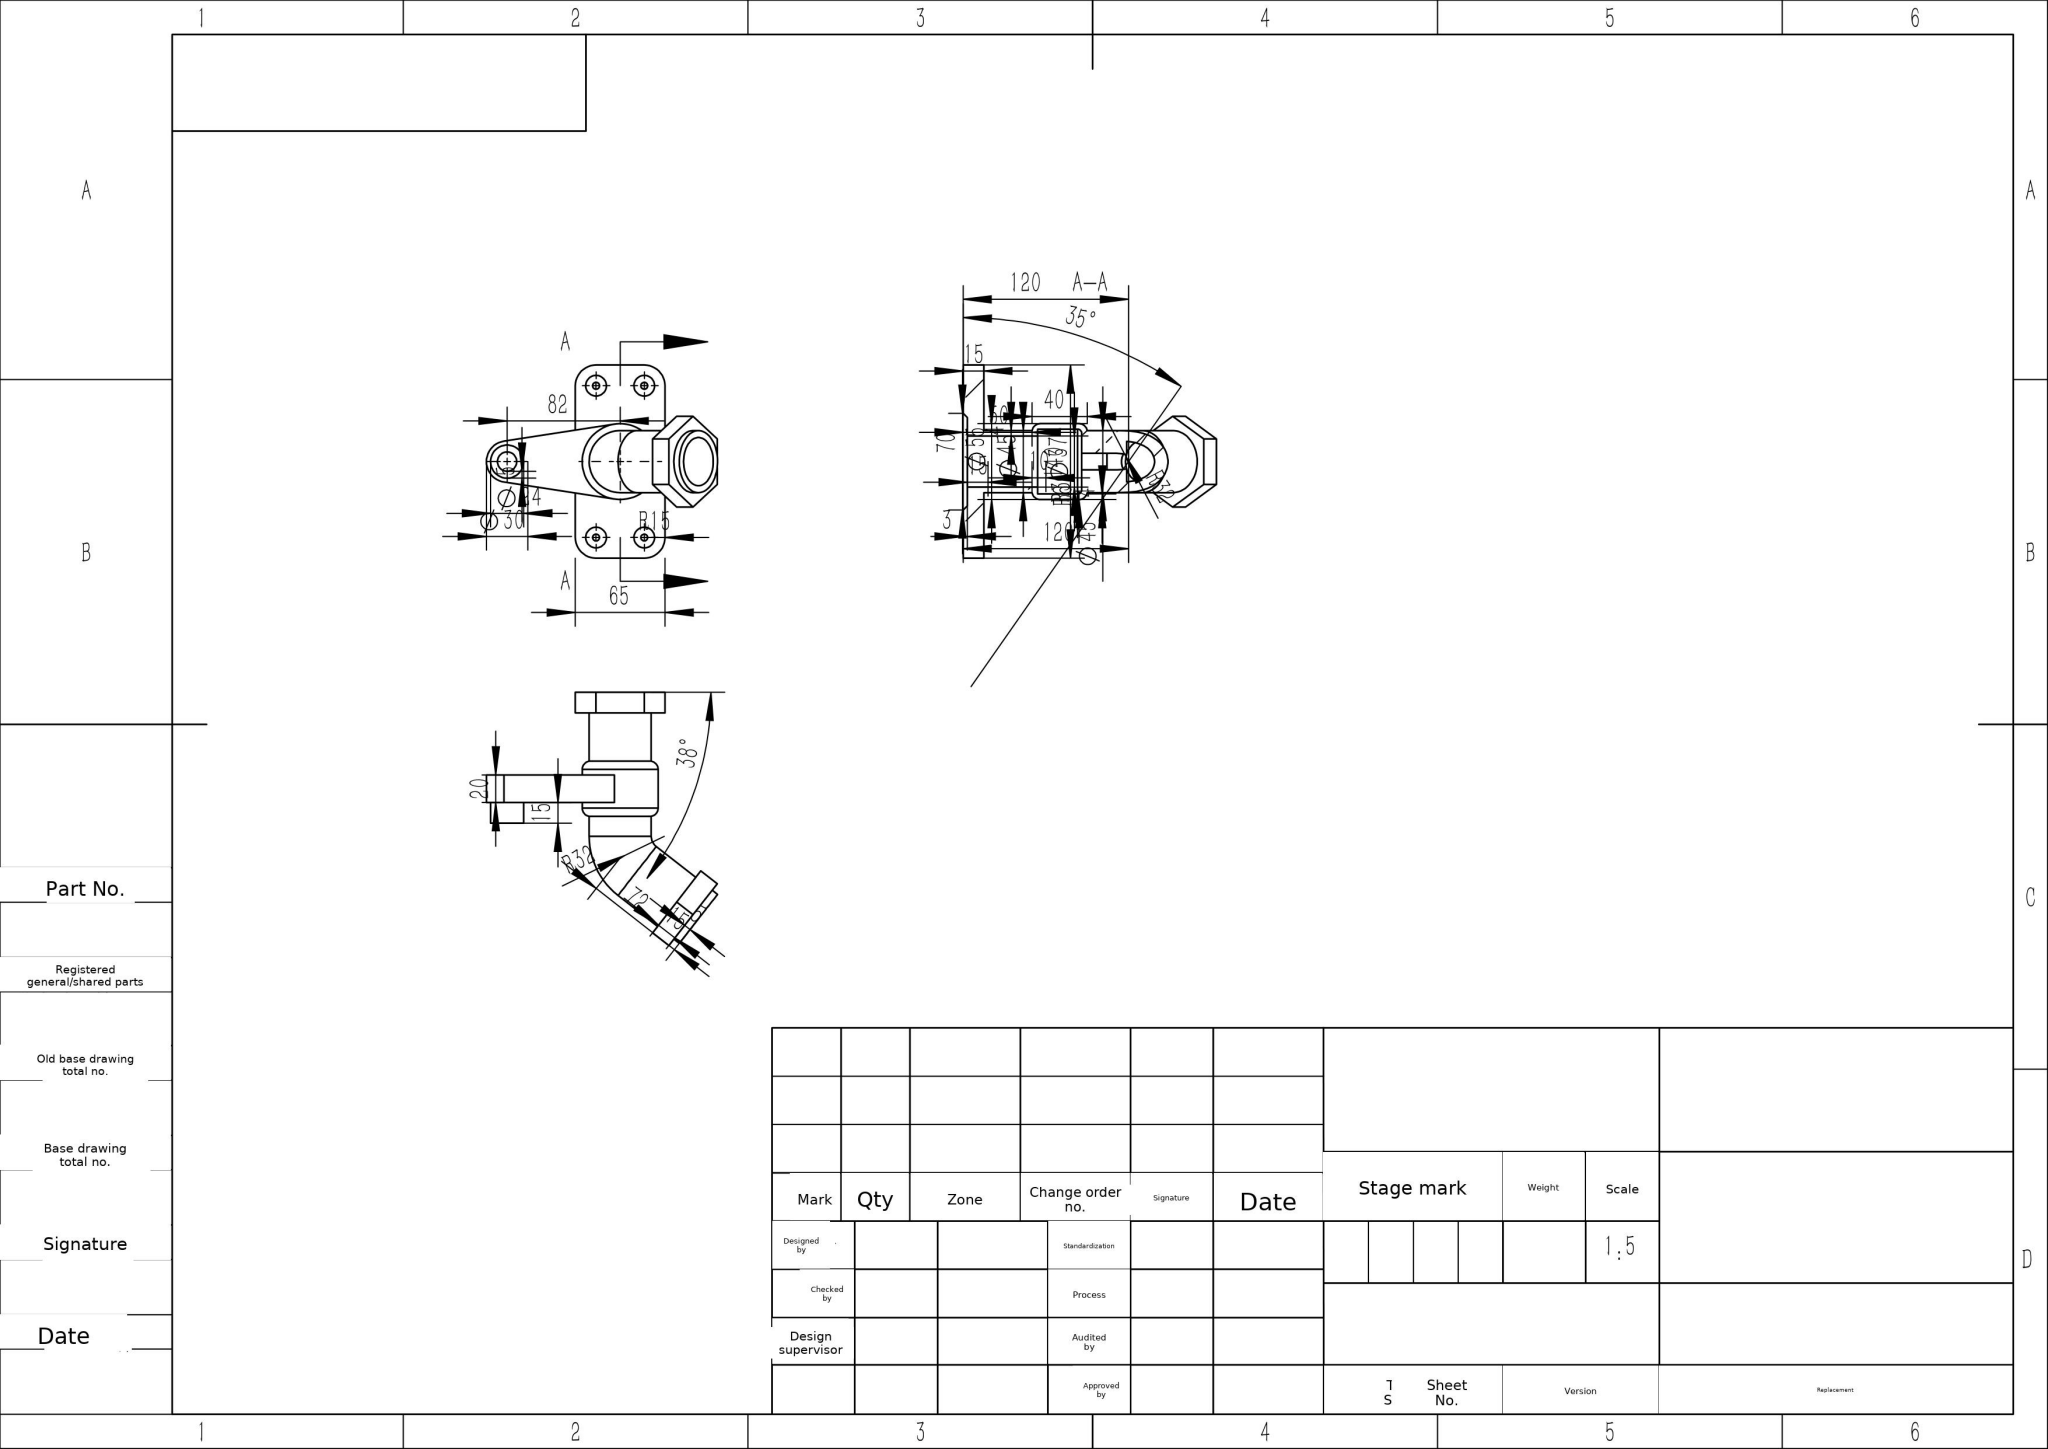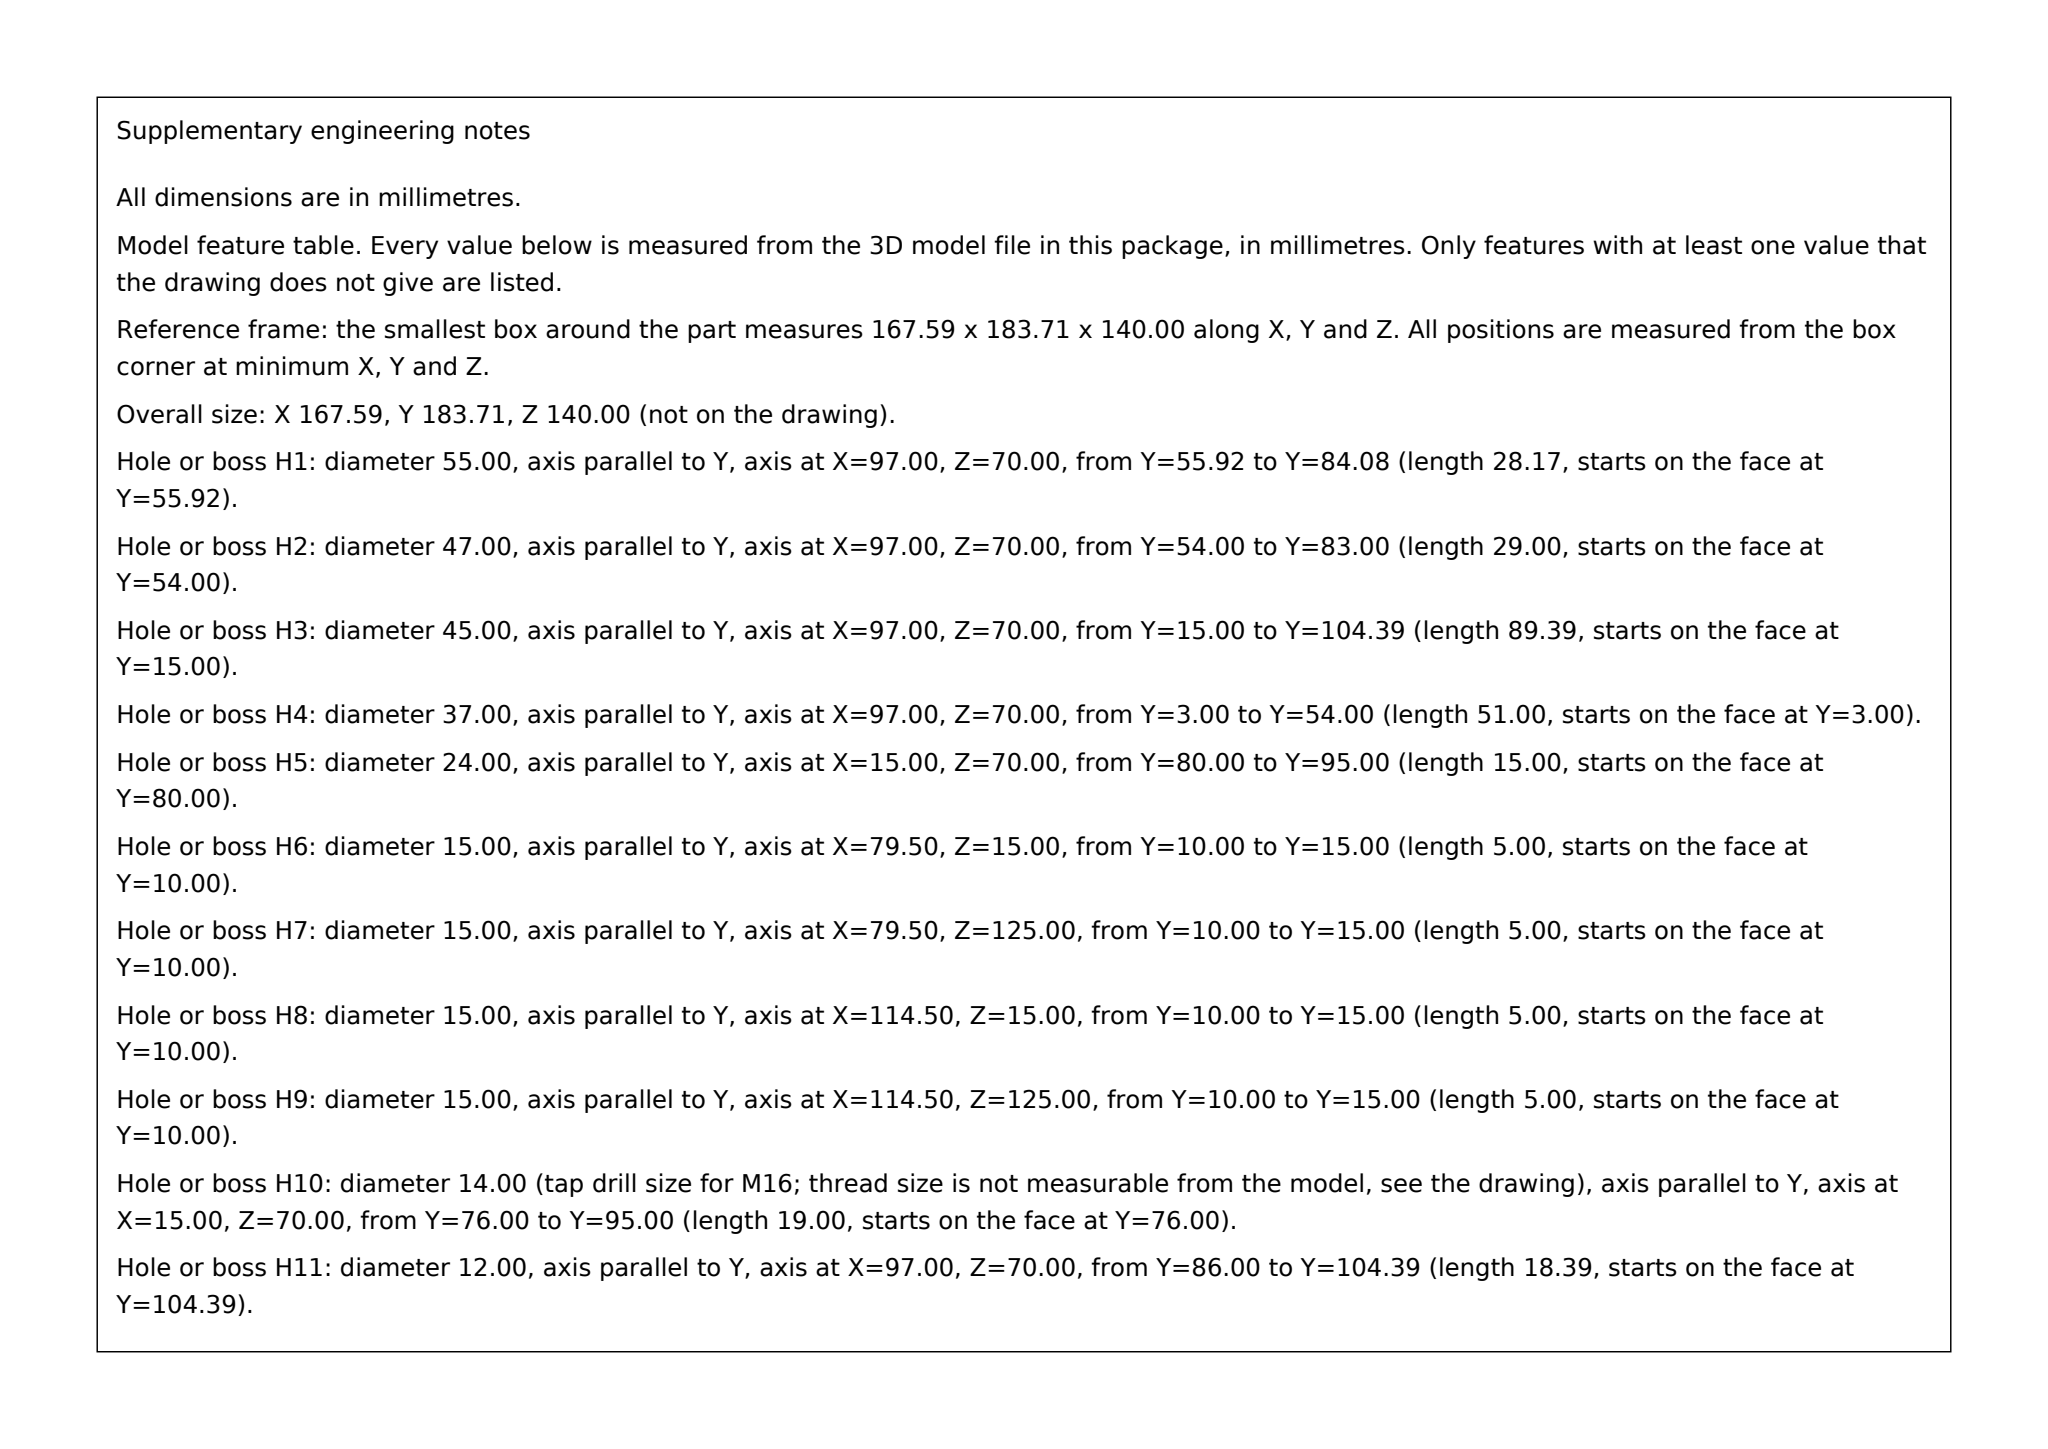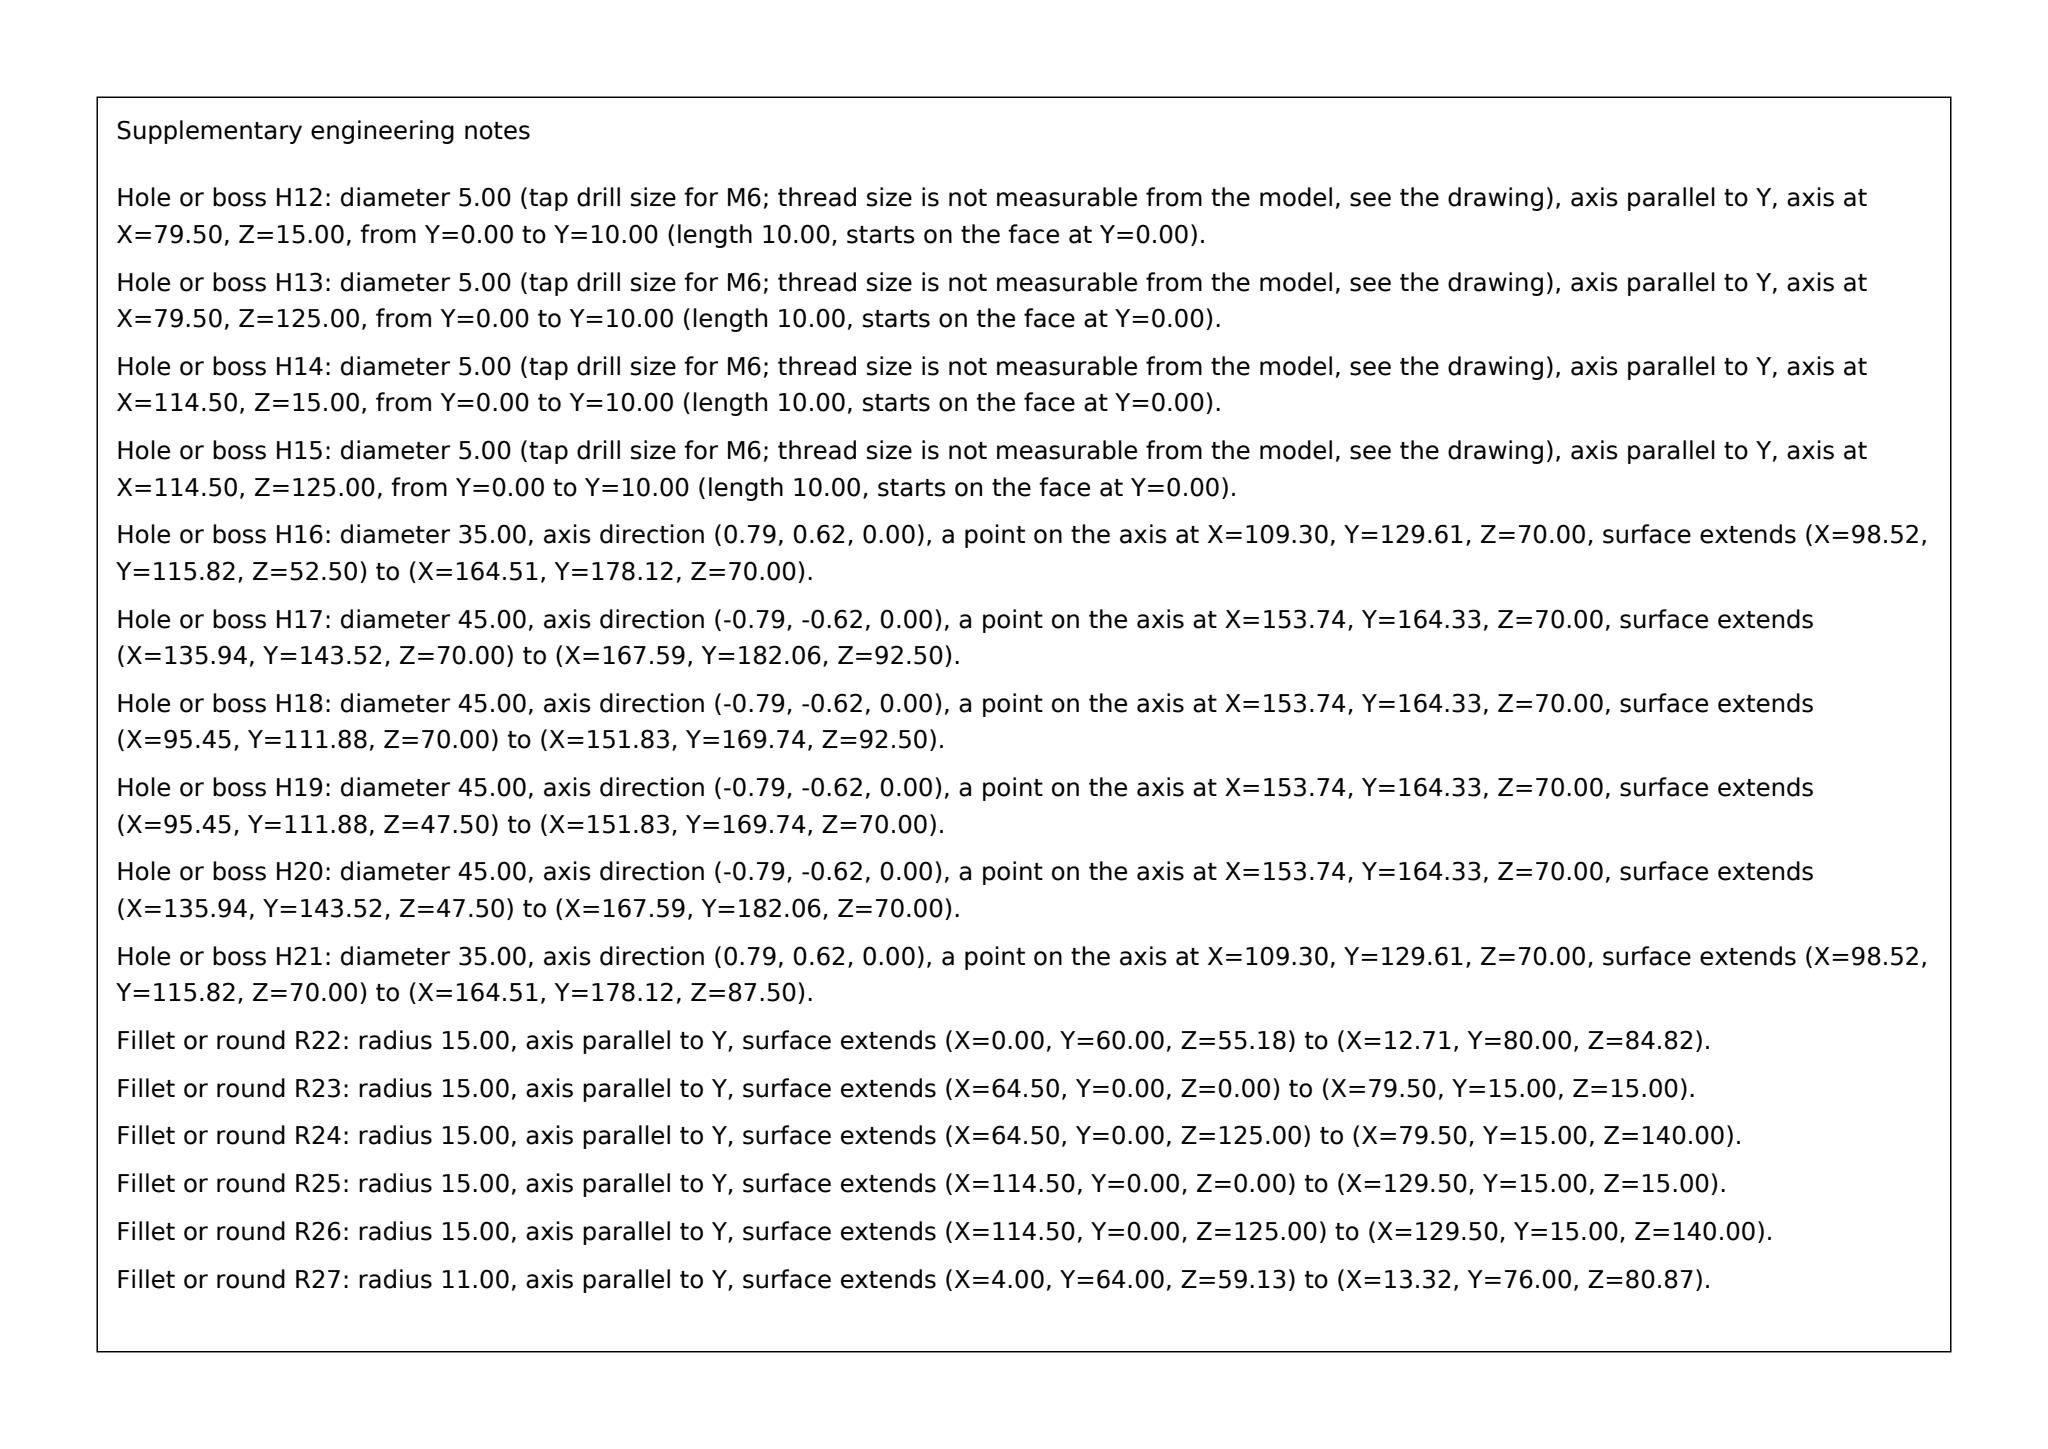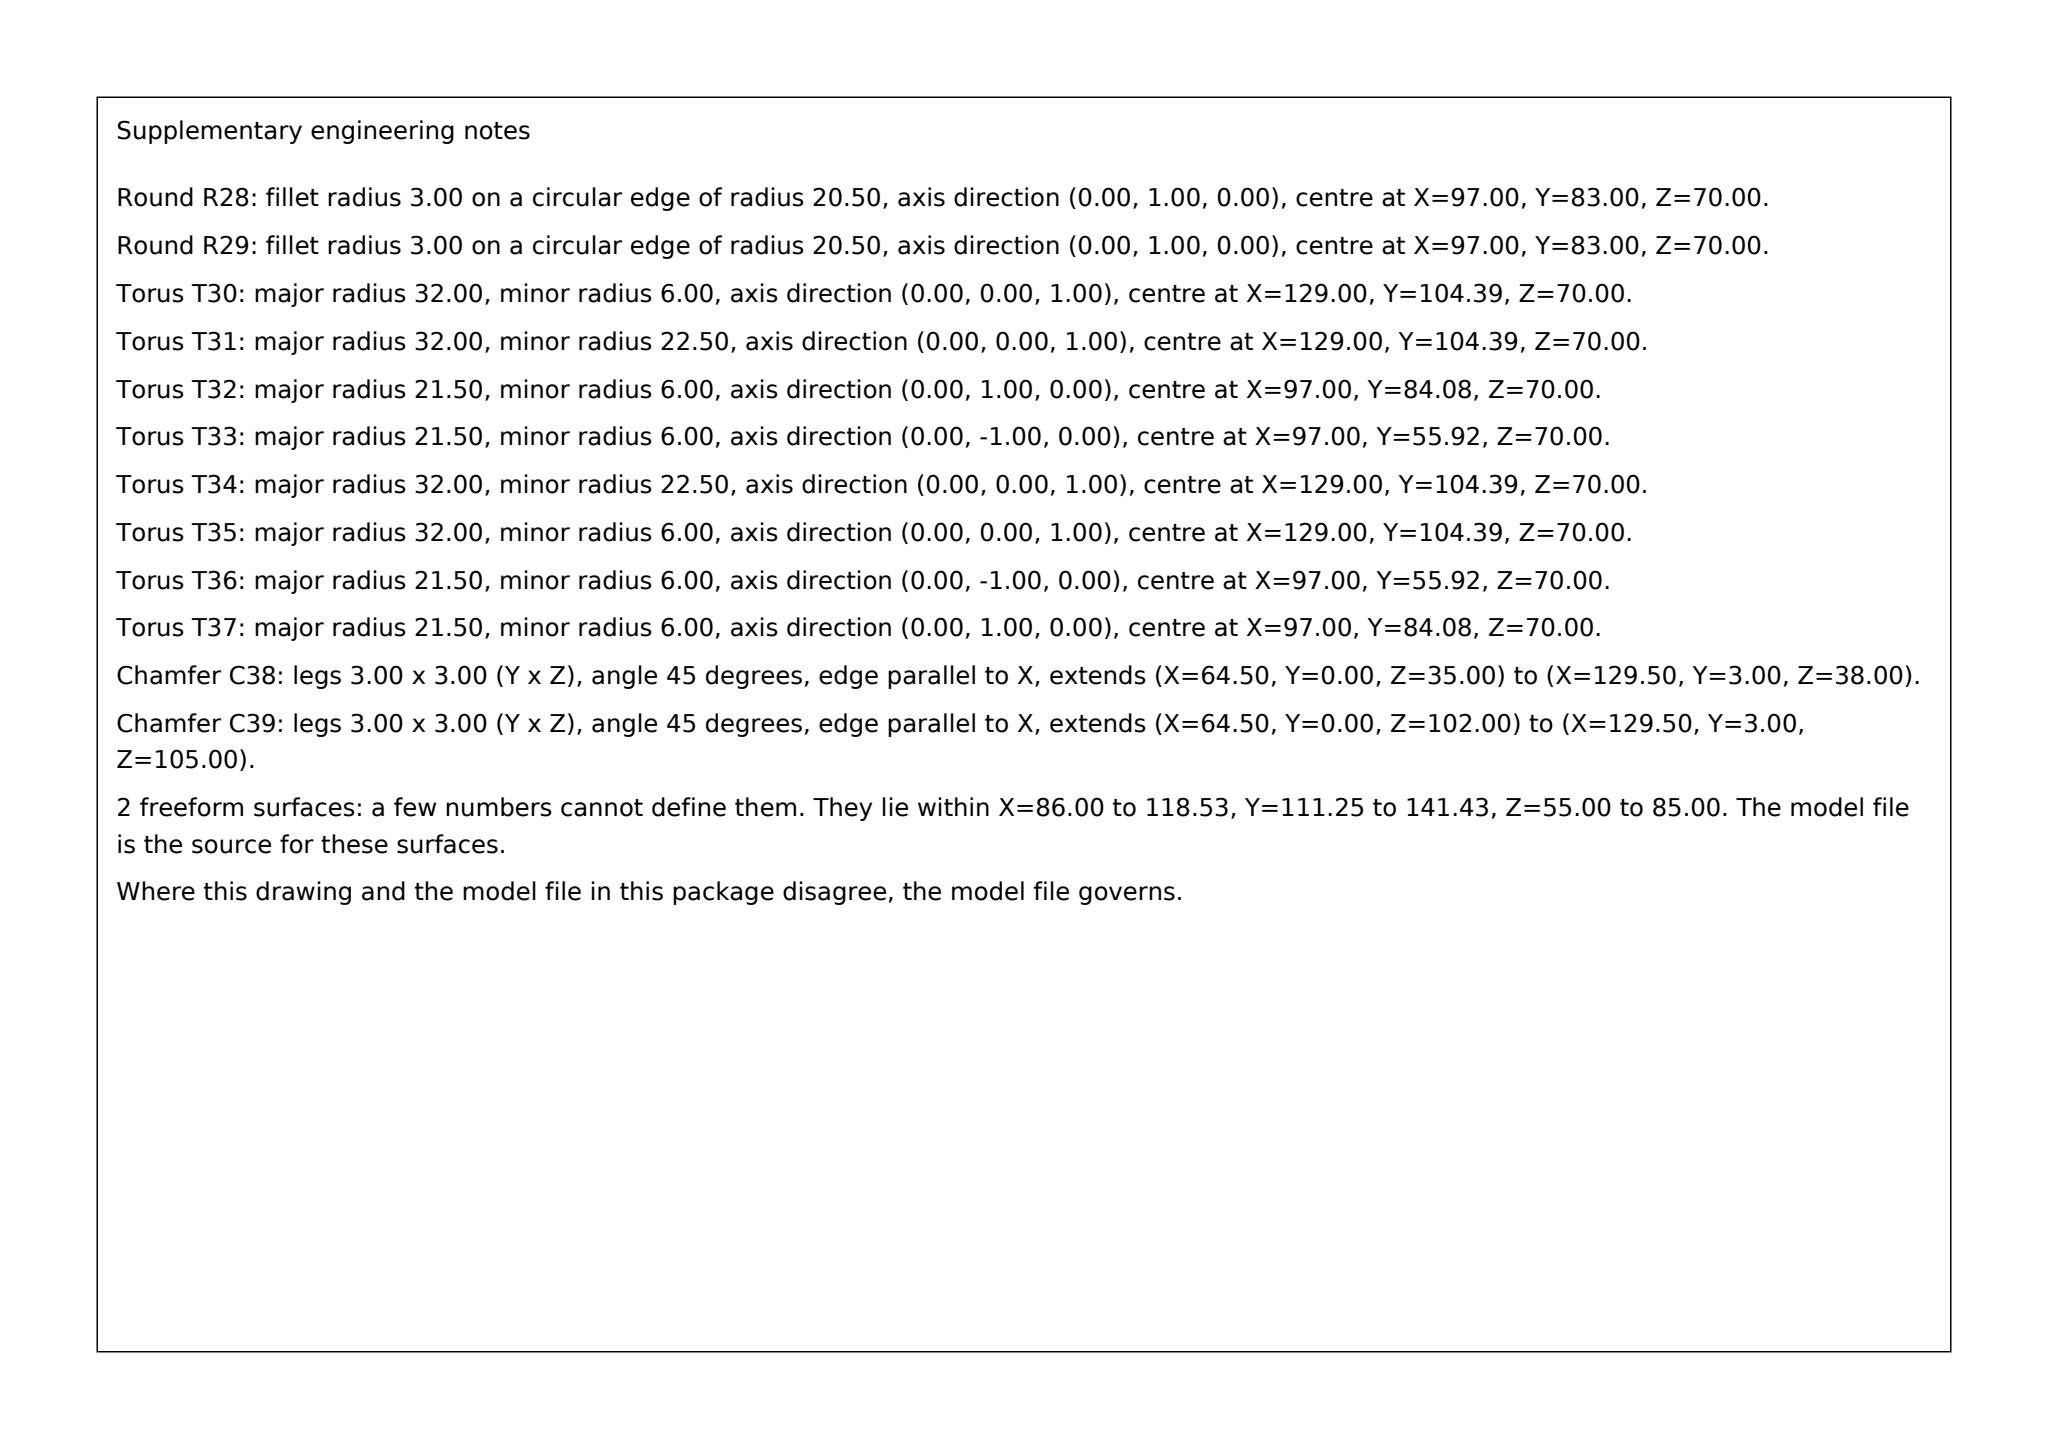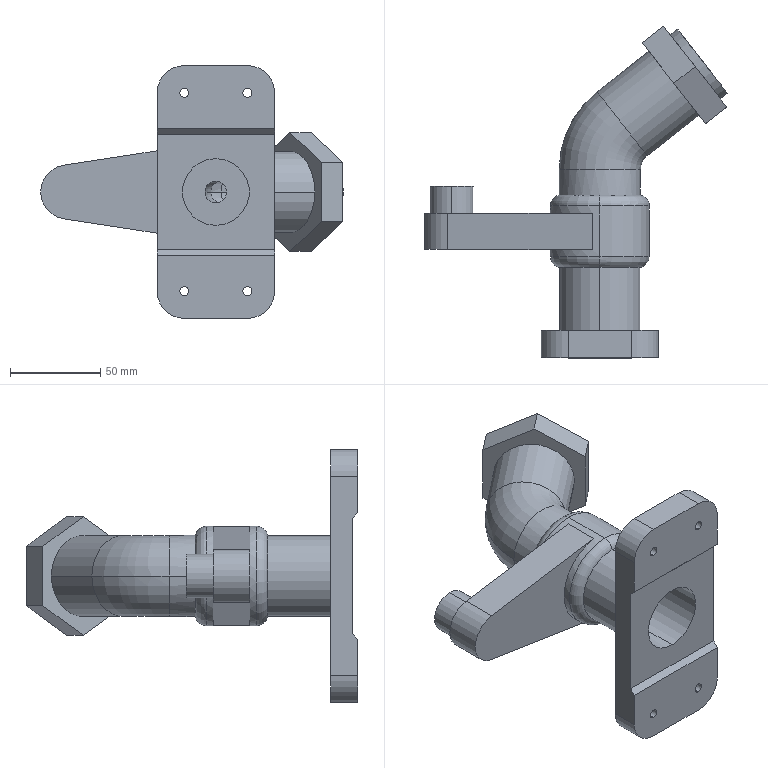Part | SolidWorks | mm | 1 solid | 92 faces | box 167.59 x 183.71 x 140 mm | volume 294053 mm3 | cylinder 44 | plane 36 | torus 10 | spline 2 | commonest cylinder face diameters 15 x8 5 x8 45 x8 30 x5 12 x2 35 x2 14 x2 24 x2